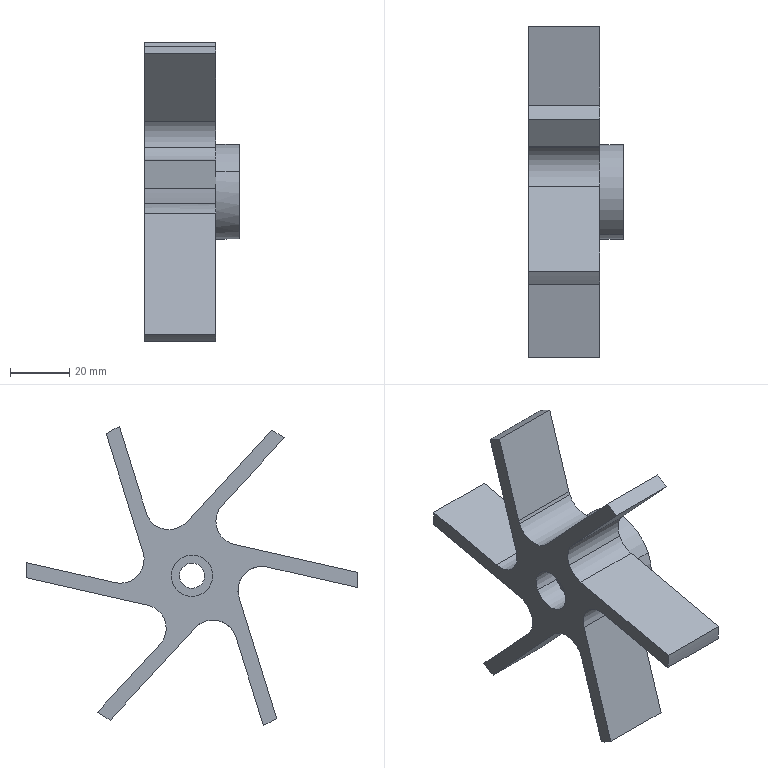Component | SolidWorks | Impeller-1 | 1 solid | 46 faces | volume 55427 mm3 | cylinder 24 | plane 22 | commonest cylinder face diameters 16 x8 112 x6 12 x4 8.5 x2 14 x2 32 x2